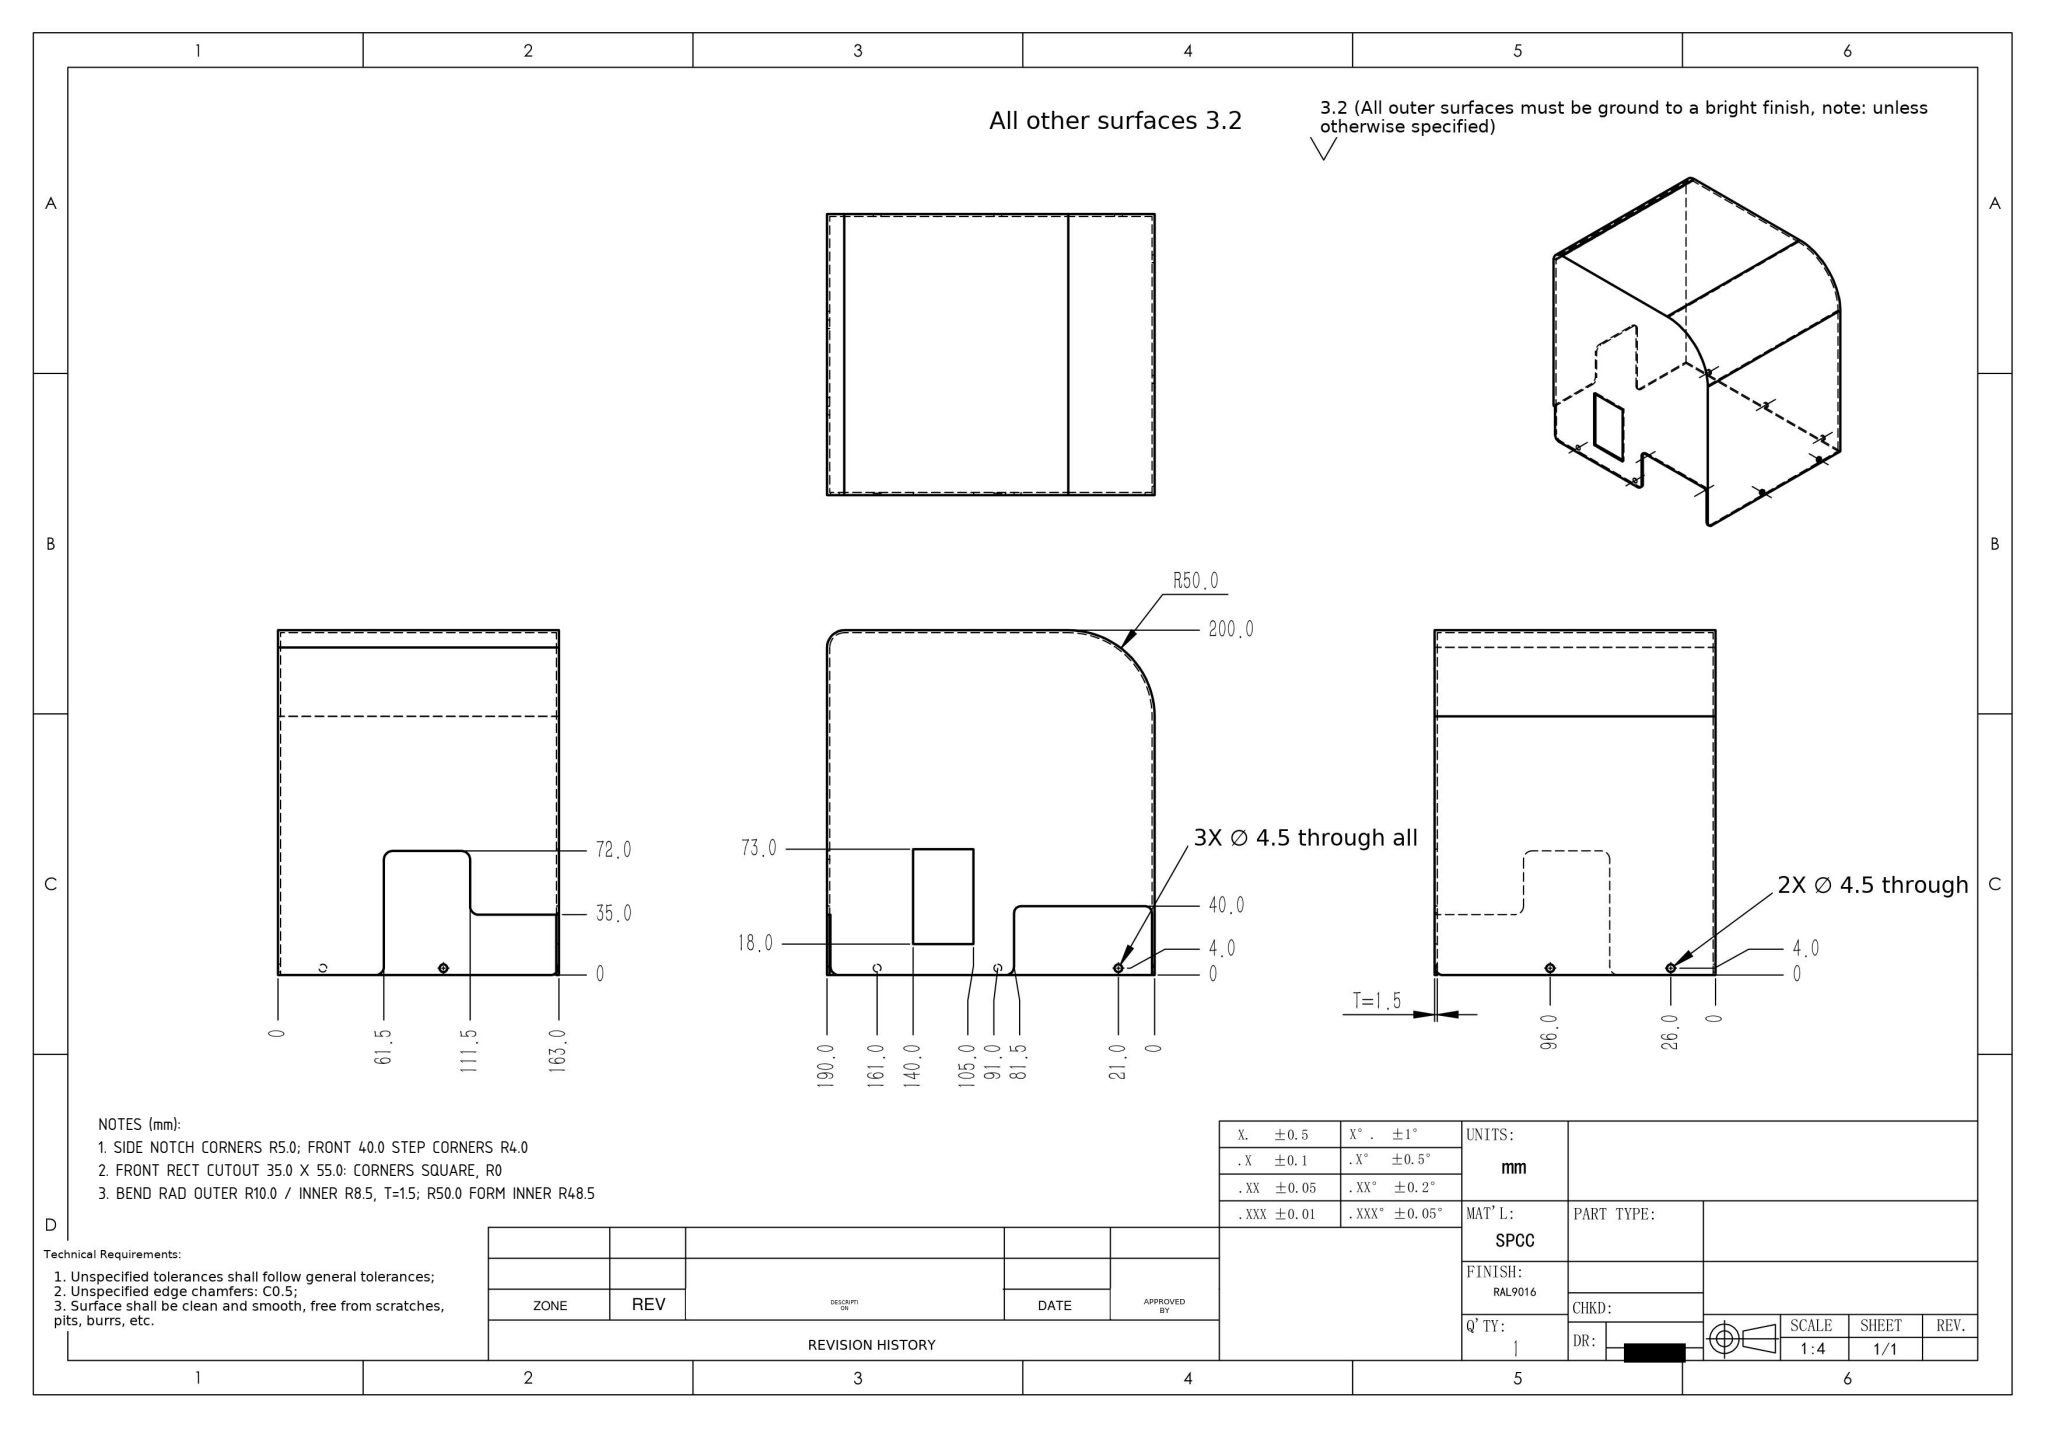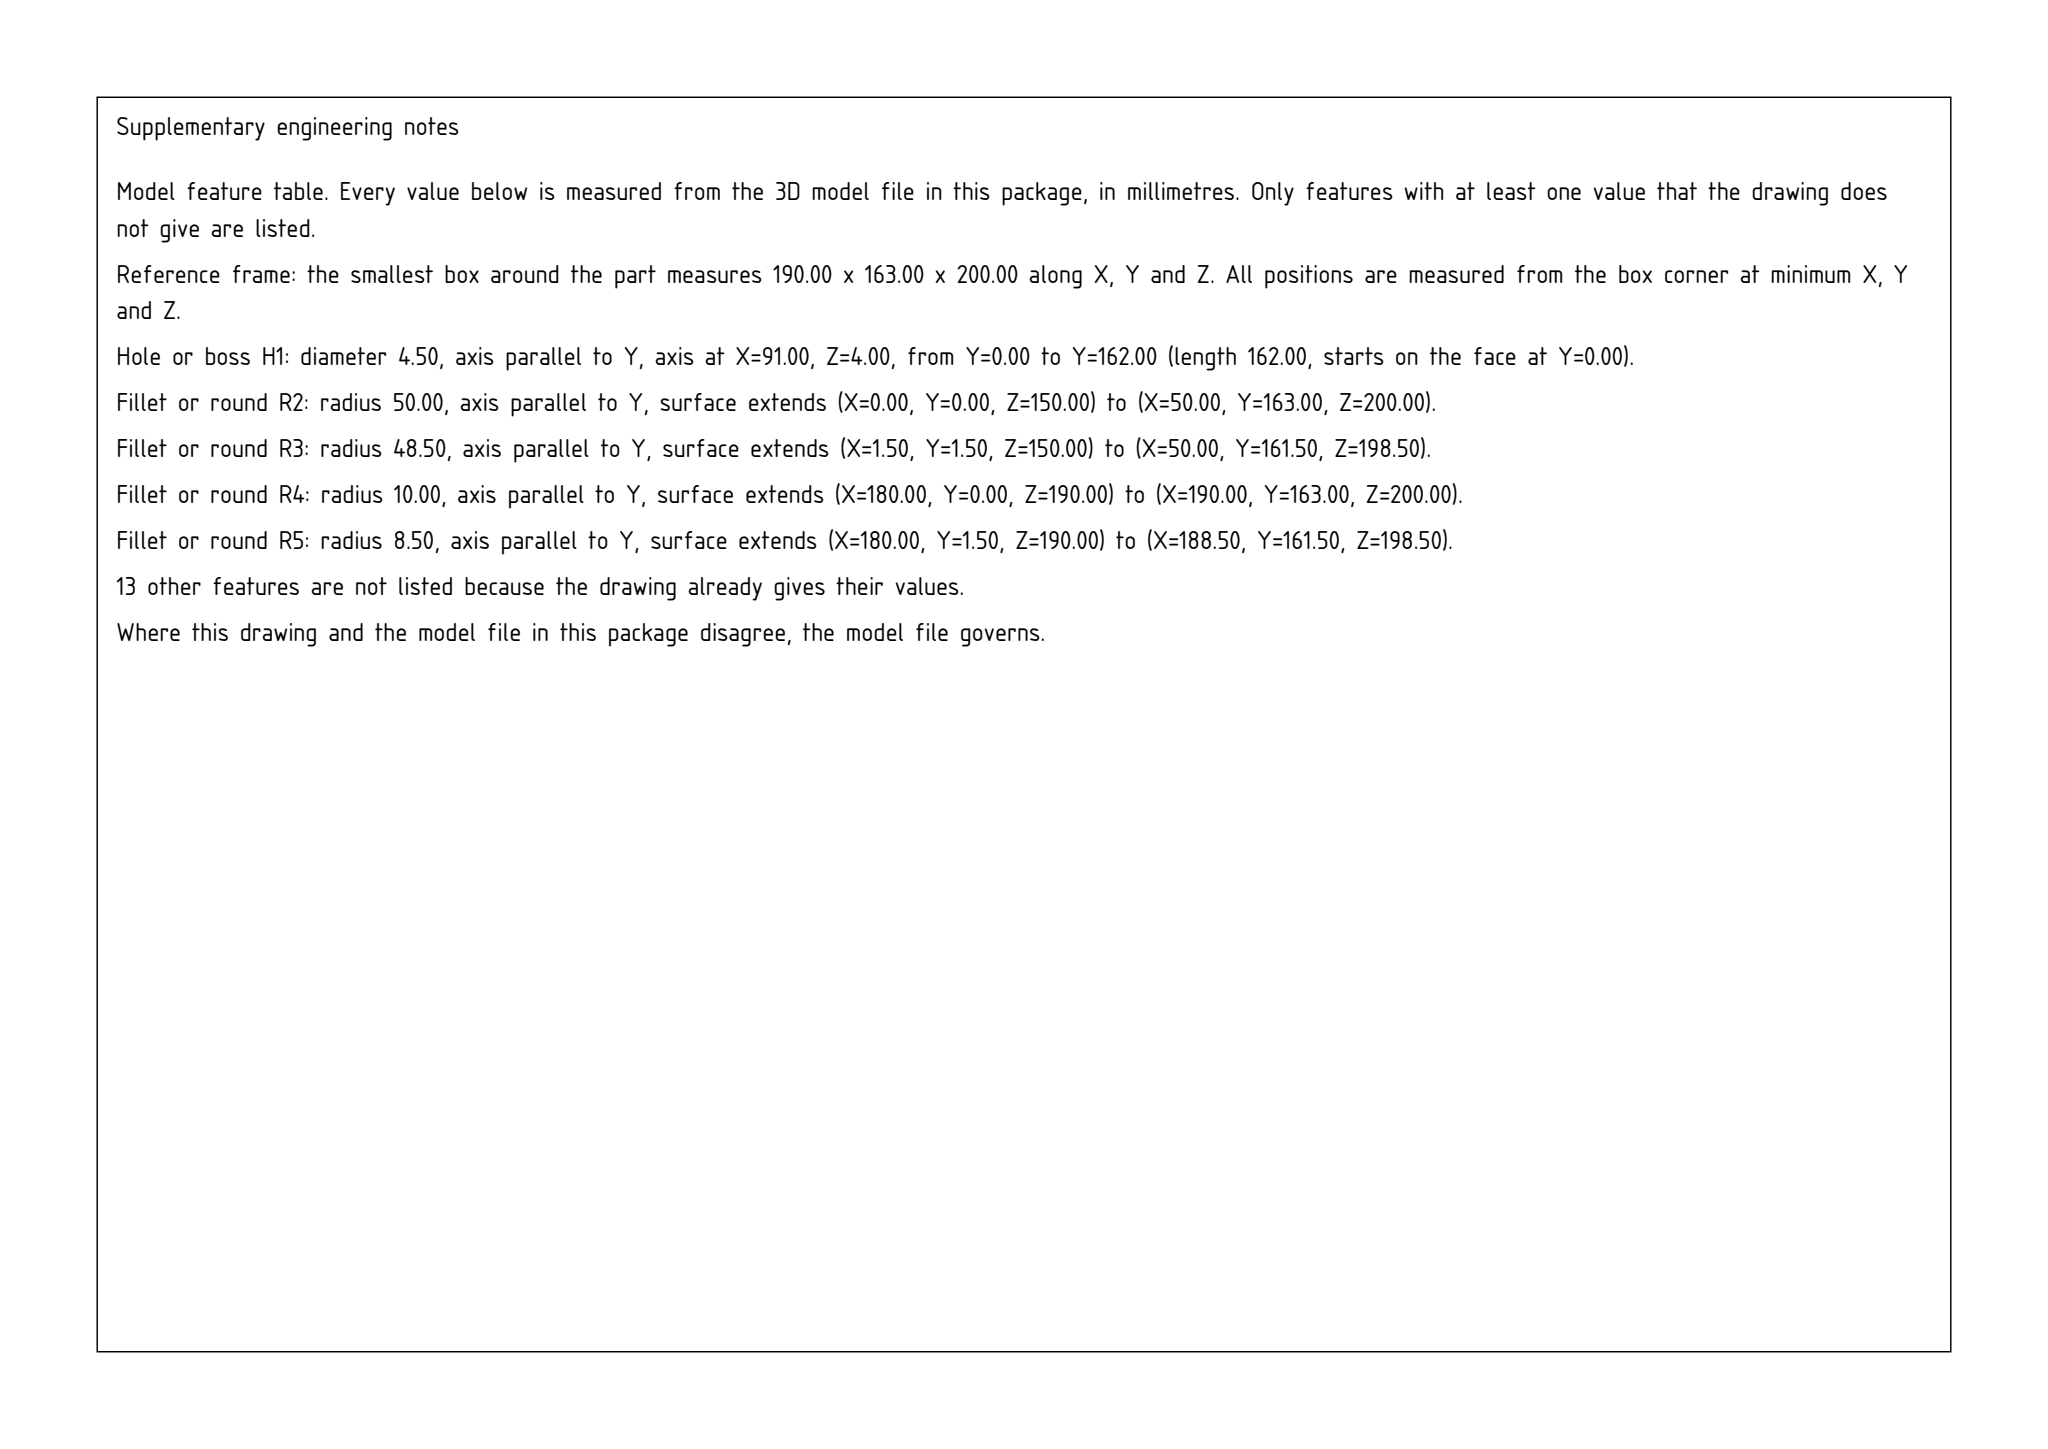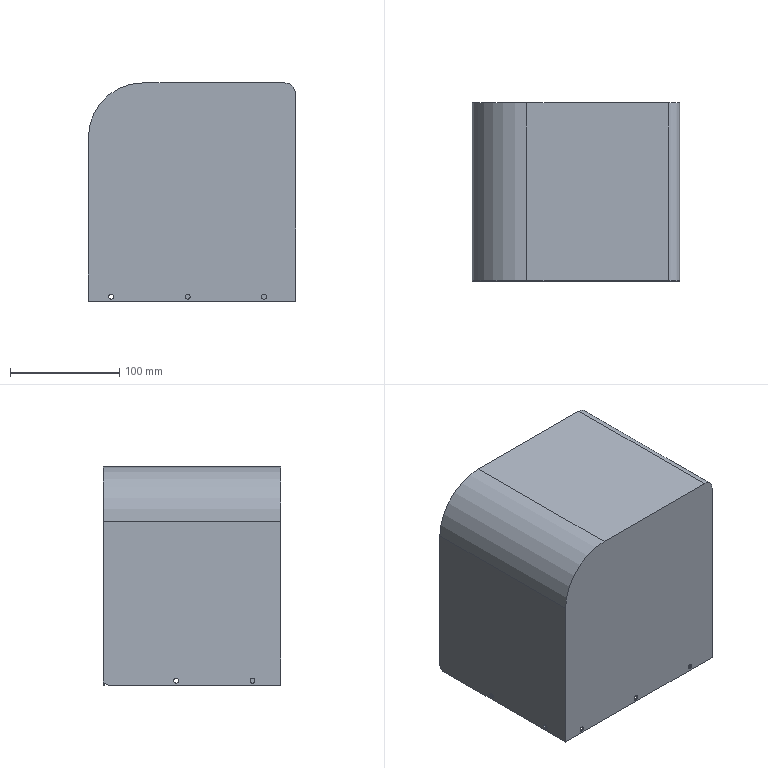Part | SolidWorks | mm | 1 solid | 52 faces | box 190 x 163 x 200 mm | volume 231214 mm3 | cylinder 27 | plane 25 | commonest cylinder face diameters 4.5 x14 10 x7 8 x2 20 x1 100 x1 17 x1 97 x1
Drawing notes:
SIDE NOTCH CORNERS R5.0; FRONT 40.0 STEP CORNERS R4.0 | from the solid: dia 10 x-axis cyls at y/z 56.5/5, 66.5/67, 106.5/67, 116.5/40, 158/5 = R5; dia 8 y-axis cyls at x/z 5.5/36, 77.5/36 = R4
FRONT RECT CUTOUT 35.0 X 55.0: CORNERS SQUARE, R0 | from the solid: x planes 105.0/140.0, z planes 18.0/73.0; no fillet radii in model
BEND RAD OUTER R10.0 / INNER R8.5, T=1.5; R50.0 FORM INNER R48.5 | from the solid: dia 20/17 y-axis cyls at [180,-,190]; dia 100/97 y-axis cyls at [50,-,150]; plane offsets 0/1.5
build123d program:
from build123d import *

# Parameters (mm, degrees)
SKETCH1_W                = 190
SKETCH1_H                = 163
BOSS_EXTRUDE1_DEPTH      = 200
FILLET3_R                = 10
FILLET1_R                = 50
SHELL1_T                 = -1.5
CUT_EXTRUDE1_REACH       = 276.944
SKETCH2_W                = 35
SKETCH2_H                = 55
CUT_EXTRUDE2_DEPTH       = 2
M4_CLEARANCE_HOLE1_D     = 4.5
M4_CLEARANCE_HOLE1_DEPTH = 1.5
M4_CLEARANCE_HOLE2_D     = 4.5
BOSS_EXTRUDE3_START      = -1
SKETCH10_R               = 2.25
BOSS_EXTRUDE3_DEPTH      = 1
FILLET2_R                = 5


with BuildPart() as part:
    # Sketch1 → Boss-Extrude1 (new body)
    with BuildSketch(Plane.XY):
        Rectangle(SKETCH1_W, SKETCH1_H)
    extrude(amount=BOSS_EXTRUDE1_DEPTH)

    # Fillet3
    fillet3_edges = [part.edges().sort_by_distance(p)[0] for p in [
        (95, 0, 200),
    ]]
    fillet(fillet3_edges, radius=FILLET3_R)

    # Fillet1
    fillet1_edges = [part.edges().sort_by_distance(p)[0] for p in [
        (-95, 0, 200),
    ]]
    fillet(fillet1_edges, radius=FILLET1_R)

    # Shell1
    shell1_openings = [part.faces().sort_by_distance(p)[0] for p in [
        (0, 0, 0),
    ]]
    offset(amount=SHELL1_T, openings=shell1_openings, kind=Kind.INTERSECTION)

    # Sketch2 → Cut-Extrude1 (cut, up to next)
    with BuildSketch(Plane.XZ.offset(-81.5), mode=Mode.PRIVATE) as cut_extrude1_sk1:
        with BuildLine():
            Line((-93.5, 0), (-13.5, 0))
            Line((-13.5, 0), (-13.5, 36))
            ThreePointArc((-13.5, 36), (-14.672, 38.828), (-17.5, 40))
            Line((-17.5, 40), (-89.5, 40))
            ThreePointArc((-89.5, 40), (-92.328, 38.828), (-93.5, 36))
            Line((-93.5, 36), (-93.5, 0))
        make_face()
    cut_extrude1_tool1 = extrude(cut_extrude1_sk1.sketch, amount=CUT_EXTRUDE1_REACH, mode=Mode.PRIVATE) & part.part
    # Sketch2 → Cut-Extrude1 (cut, up to next)
    with BuildSketch(Plane.XZ.offset(-81.5), mode=Mode.PRIVATE) as cut_extrude1_sk2:
        with Locations((27.5, 45.5)):
            Rectangle(SKETCH2_W, SKETCH2_H)
    cut_extrude1_tool2 = extrude(cut_extrude1_sk2.sketch, amount=CUT_EXTRUDE1_REACH, mode=Mode.PRIVATE) & part.part
    add(cut_extrude1_tool1.solids().sort_by_distance((-53.5, 81.5, 19.959))[0], mode=Mode.SUBTRACT)
    add(cut_extrude1_tool2.solids().sort_by_distance((27.5, 81.5, 45.5))[0], mode=Mode.SUBTRACT)

    # Sketch5 → Cut-Extrude2 (cut)
    with BuildSketch(Plane(origin=(95, 0, 0), x_dir=(0, 0, -1), z_dir=(1, 0, 0))):
        Polygon((0, -20), (-72, -20), (-72, 30), (-35, 30), (-35, 81.5), (0, 81.5), align=None)
    extrude(amount=-CUT_EXTRUDE2_DEPTH, mode=Mode.SUBTRACT)

    # M4 Clearance Hole1
    with Locations(Plane.ZY.offset(95)):
        with Locations((4, 14.5), (4, -55.5)):
            Hole(M4_CLEARANCE_HOLE1_D / 2, depth=M4_CLEARANCE_HOLE1_DEPTH)

    # M4 Clearance Hole2 (through all)
    with Locations(Plane(origin=(0, 81.5, 0), x_dir=(1, 0, 0), z_dir=(0, 1, 0))):
        with Locations((-74, -4), (-4, -4), (66, -4)):
            Hole(M4_CLEARANCE_HOLE2_D / 2)

    # Sketch10 → Boss-Extrude3 (add)
    with BuildSketch(Plane(origin=(0, 81.5, 0), x_dir=(1, 0, 0), z_dir=(0, 1, 0)).offset(BOSS_EXTRUDE3_START)):
        with Locations(Location((-4, -4, 0), (0, 0, 270))):
            Circle(SKETCH10_R)
        with Locations(Location((66, -4, 0), (0, 0, 270))):
            Circle(SKETCH10_R)
    extrude(amount=BOSS_EXTRUDE3_DEPTH)

    # Fillet2
    fillet2_edges = [part.edges().sort_by_distance(p)[0] for p in [
        (94.25, 30, 72),
        (94.25, -20, 72),
        (93, 80.75, 0),
        (94.25, 30, 35),
        (94.25, -20, 0),
        (-13.5, 80.75, 0),
        (-94.25, 81.5, 0),
    ]]
    fillet(fillet2_edges, radius=FILLET2_R)


solid = part.part